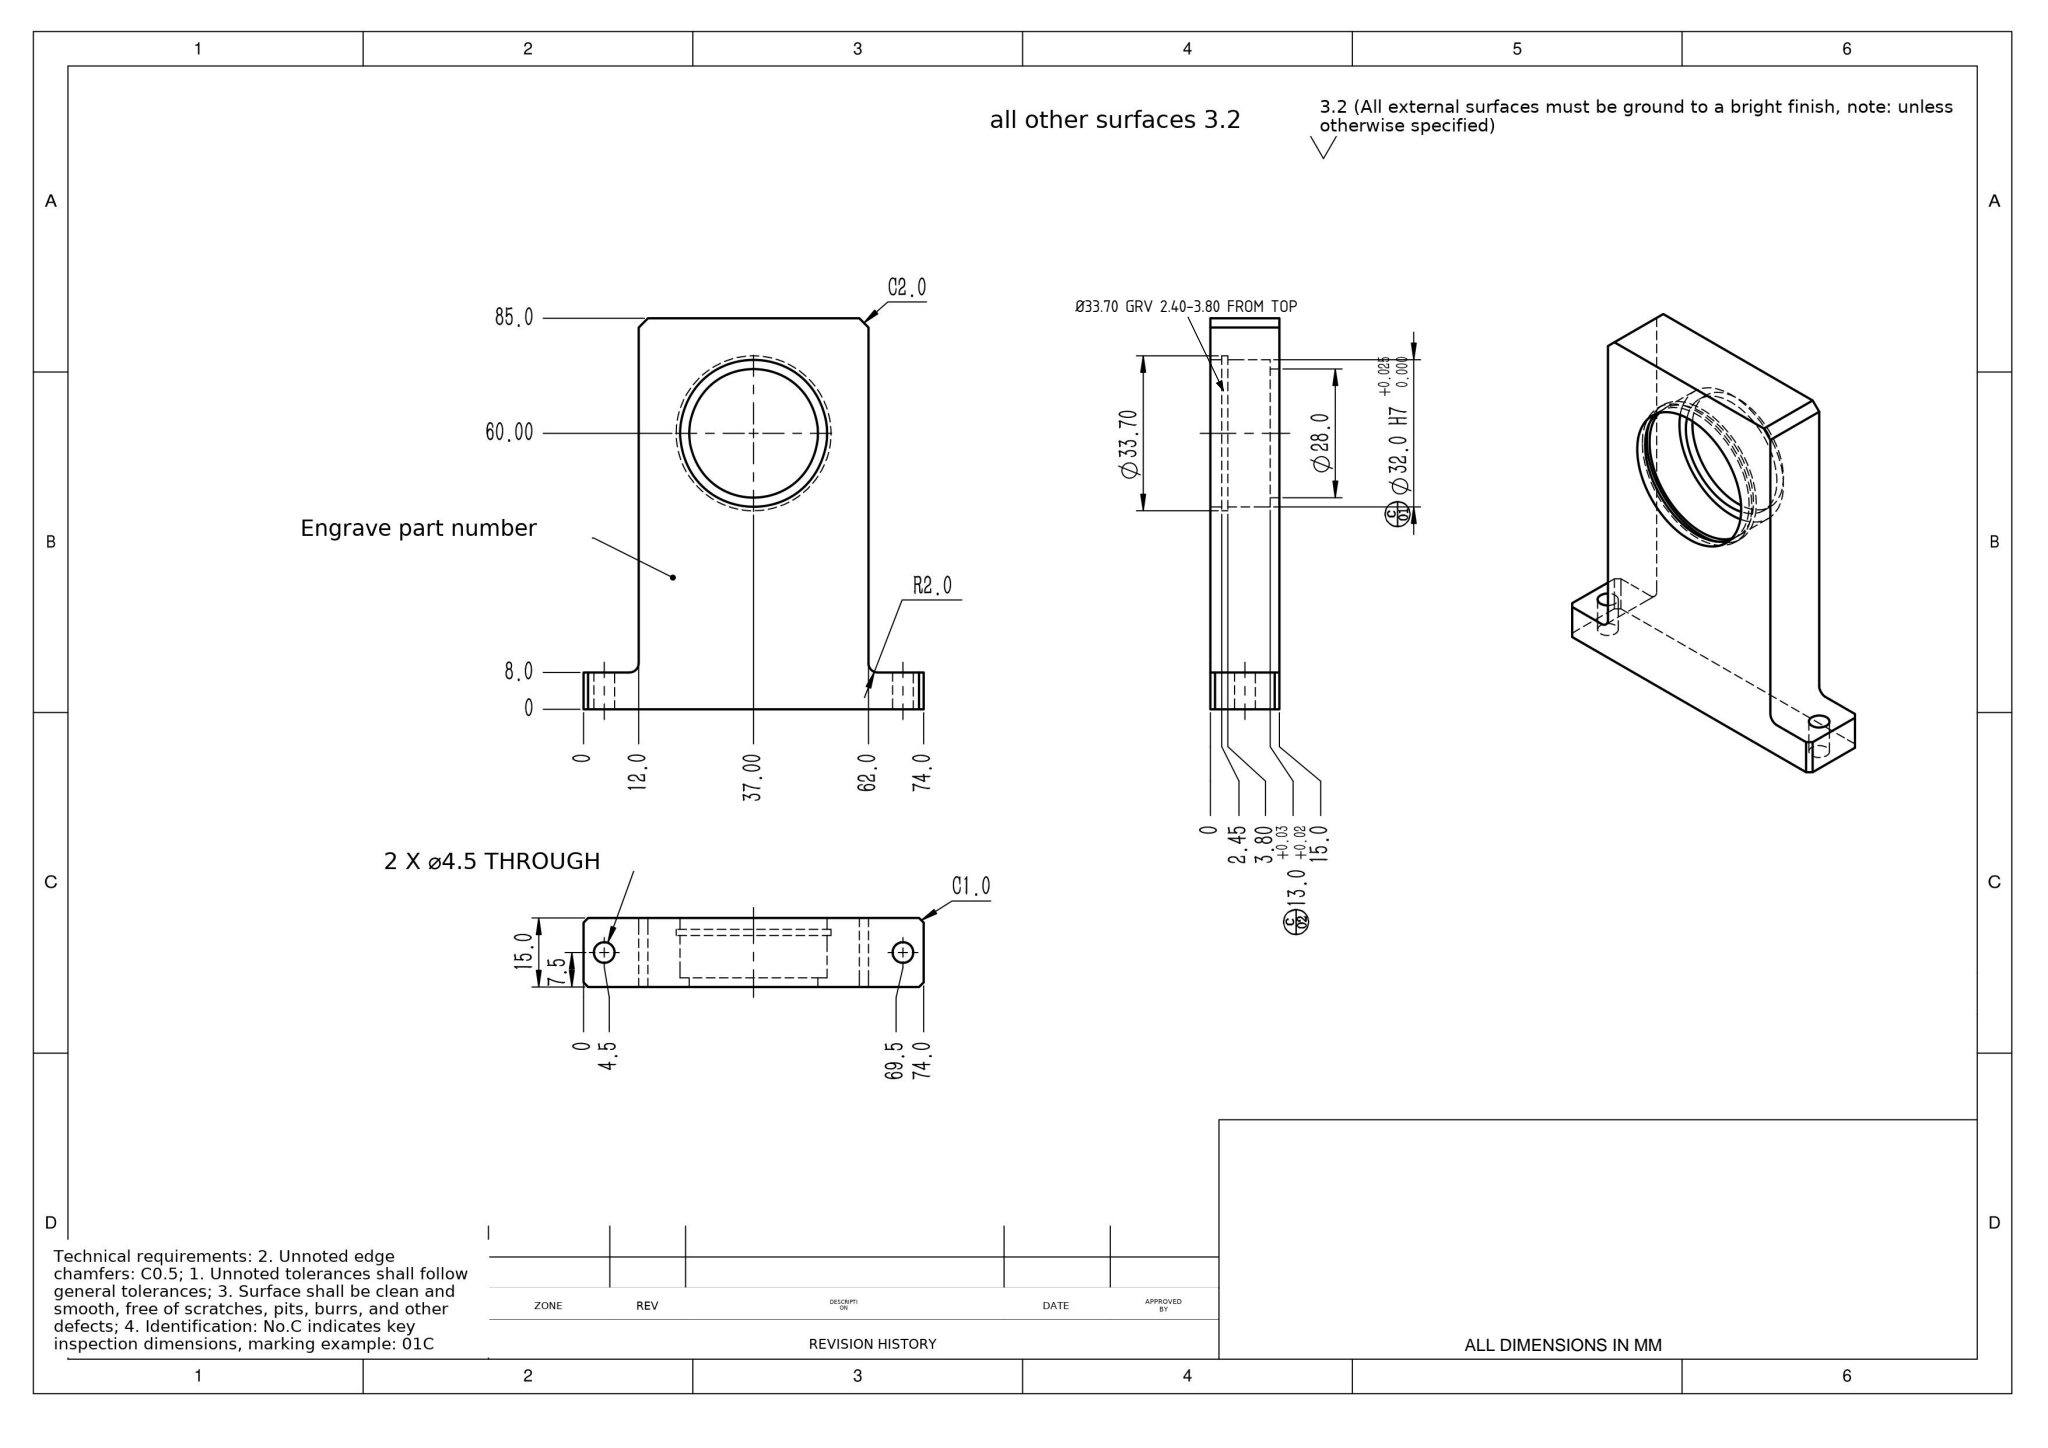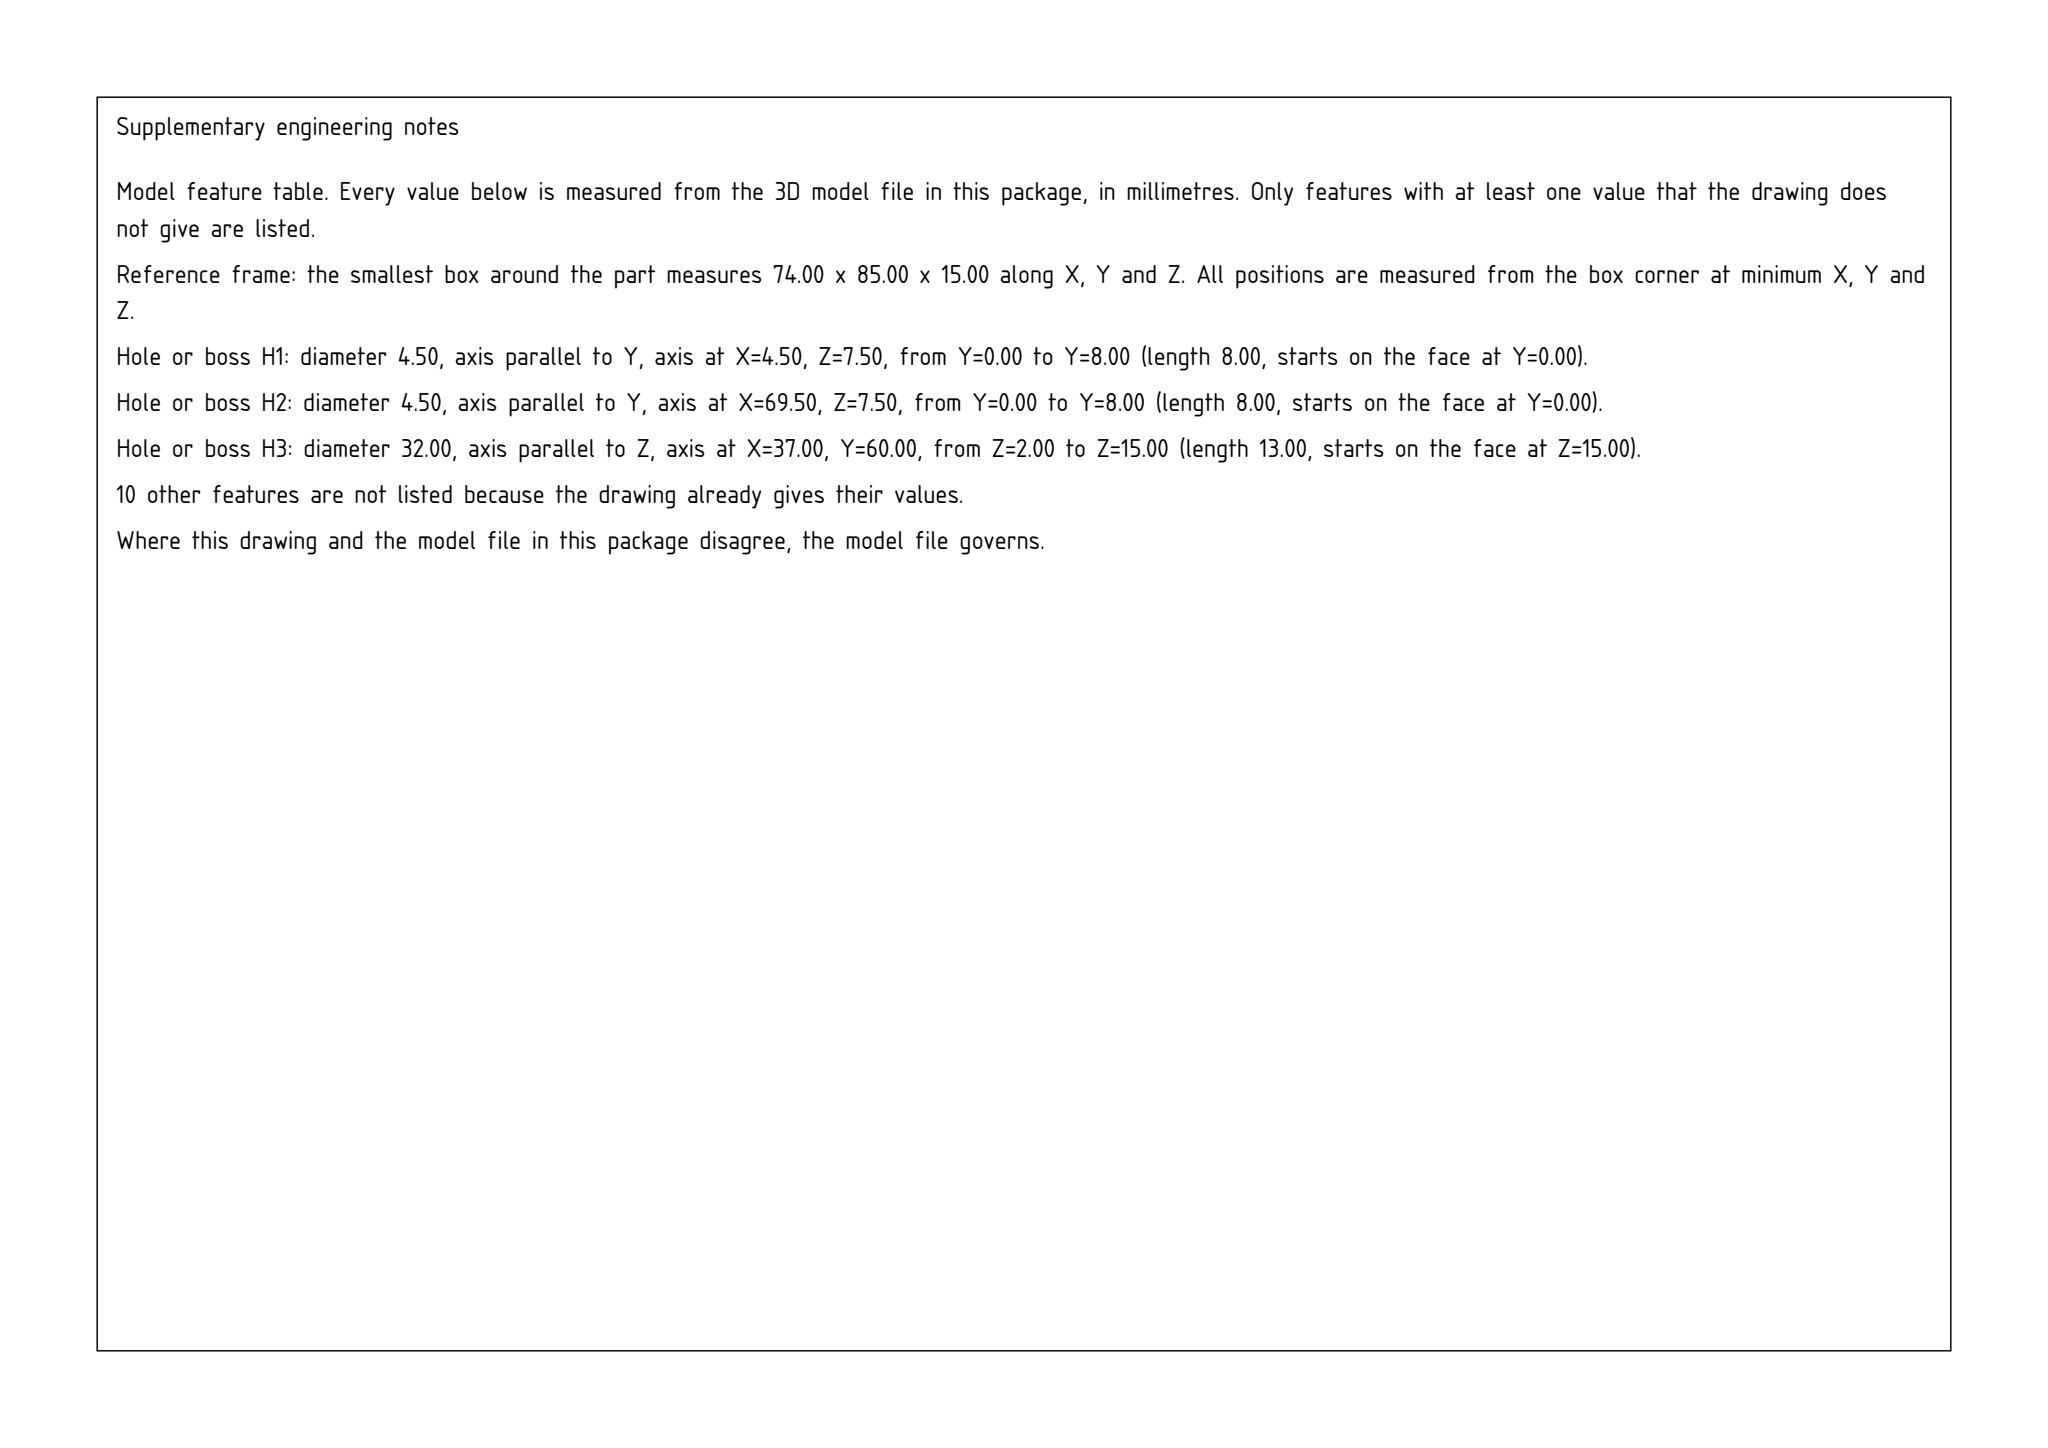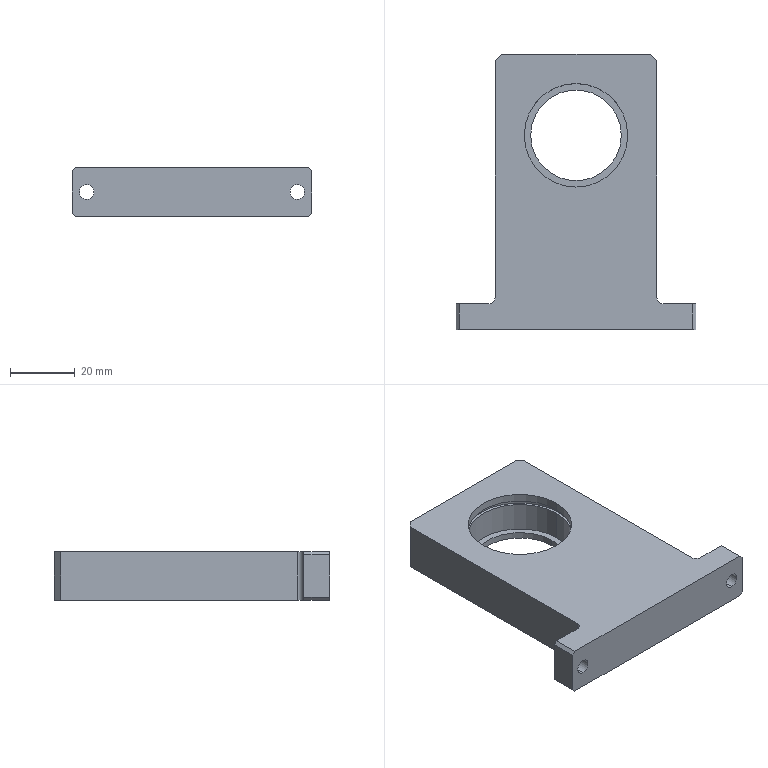Part | SolidWorks | mm | 1 solid | 33 faces | box 74 x 85 x 15 mm | volume 54520 mm3 | plane 19 | cylinder 14 | commonest cylinder face diameters 4.5 x4 32 x4 33.7 x2 28 x2 4 x2
Drawing notes:
SIDE VIEW ORD: Ø33.70 GRV 2.40 TO 3.80 FROM TOP; 15.0 OVERALL THK | from the solid: Bore Ø33.70 spans z 11.2-12.6; top face z=15.0 -> 2.40 and 3.80 from top; part thickness z 0-15.0
build123d program:
from build123d import *

# Parameters (mm, degrees)
BOSS_EXTRUDE1_DEPTH = 7.5
SKETCH2_R           = 16
CUT_EXTRUDE1_DEPTH  = 94.91
BOSS_EXTRUDE2_START = -2
SKETCH3_R           = 16
SKETCH3_R_2         = 14
BOSS_EXTRUDE2_DEPTH = 2
CHAMFER1_SIZE       = 2
FILLET1_R           = 2
SKETCH4_W           = 1.35
SKETCH4_H           = 0.85
SKETCH5_R           = 2.25
CUT_EXTRUDE2_DEPTH  = 86.757
CHAMFER2_SIZE       = 1


with BuildPart() as part:
    # Sketch1 → Boss-Extrude1 (new, symmetric)
    with BuildSketch(Plane.XY):
        Polygon((-25, 0), (25, 0), (25, -77), (37, -77), (37, -85), (-37, -85), (-37, -77), (-25, -77), align=None)
    extrude(amount=BOSS_EXTRUDE1_DEPTH, both=True)

    # Sketch2 → Cut-Extrude1 (cut, through all)
    with BuildSketch(Plane.XY.offset(7.5)):
        with Locations((0, -25)):
            Circle(SKETCH2_R)
    extrude(amount=-CUT_EXTRUDE1_DEPTH, mode=Mode.SUBTRACT)

    # Sketch3 → Boss-Extrude2 (add)
    with BuildSketch(Plane(origin=(0, 0, -7.5), x_dir=(-1, 0, 0), z_dir=(0, 0, -1)).offset(BOSS_EXTRUDE2_START)):
        with Locations(Location((0, -25, 0), (0, 0, 180))):
            Circle(SKETCH3_R)
        with Locations((0, -25)):
            Circle(SKETCH3_R_2, mode=Mode.SUBTRACT)
    extrude(amount=BOSS_EXTRUDE2_DEPTH)

    # Chamfer1
    chamfer1_edges = [part.edges().sort_by_distance(p)[0] for p in [
        (-25, 0, 0),
        (25, 0, 0),
    ]]
    chamfer(chamfer1_edges, length=CHAMFER1_SIZE)

    # Fillet1
    fillet1_edges = [part.edges().sort_by_distance(p)[0] for p in [
        (25, -77, 0),
        (-25, -77, 0),
    ]]
    fillet(fillet1_edges, radius=FILLET1_R)

    # Sketch4 → Cut-Revolve1 (revolve, cut)
    with BuildSketch(Plane(origin=(0, 0, 0), x_dir=(0, 0, -1), z_dir=(1, 0, 0)), mode=Mode.PRIVATE) as cut_revolve1_sk:
        with Locations((-4.375, -8.575)):
            Rectangle(SKETCH4_W, SKETCH4_H)
    revolve(cut_revolve1_sk.sketch.rotate(Axis((0, -25, -5.5), (0, 0, 1)), 90), axis=Axis((0, -25, -5.5), (0, 0, 1)), mode=Mode.SUBTRACT)

    # Sketch5 → Cut-Extrude2 (cut, through all)
    with BuildSketch(Plane(origin=(0, -77, 0), x_dir=(1, 0, 0), z_dir=(0, 1, 0))):
        with Locations(Location((-32.5, 0, 0), (0, 0, 270))):
            Circle(SKETCH5_R)
        with Locations(Location((32.5, 0, 0), (0, 0, 270))):
            Circle(SKETCH5_R)
    extrude(amount=-CUT_EXTRUDE2_DEPTH, mode=Mode.SUBTRACT)

    # Chamfer2
    chamfer2_edges = [part.edges().sort_by_distance(p)[0] for p in [
        (-37, -81, 7.5),
        (37, -81, 7.5),
        (37, -81, -7.5),
        (-37, -81, -7.5),
    ]]
    chamfer(chamfer2_edges, length=CHAMFER2_SIZE)


solid = part.part